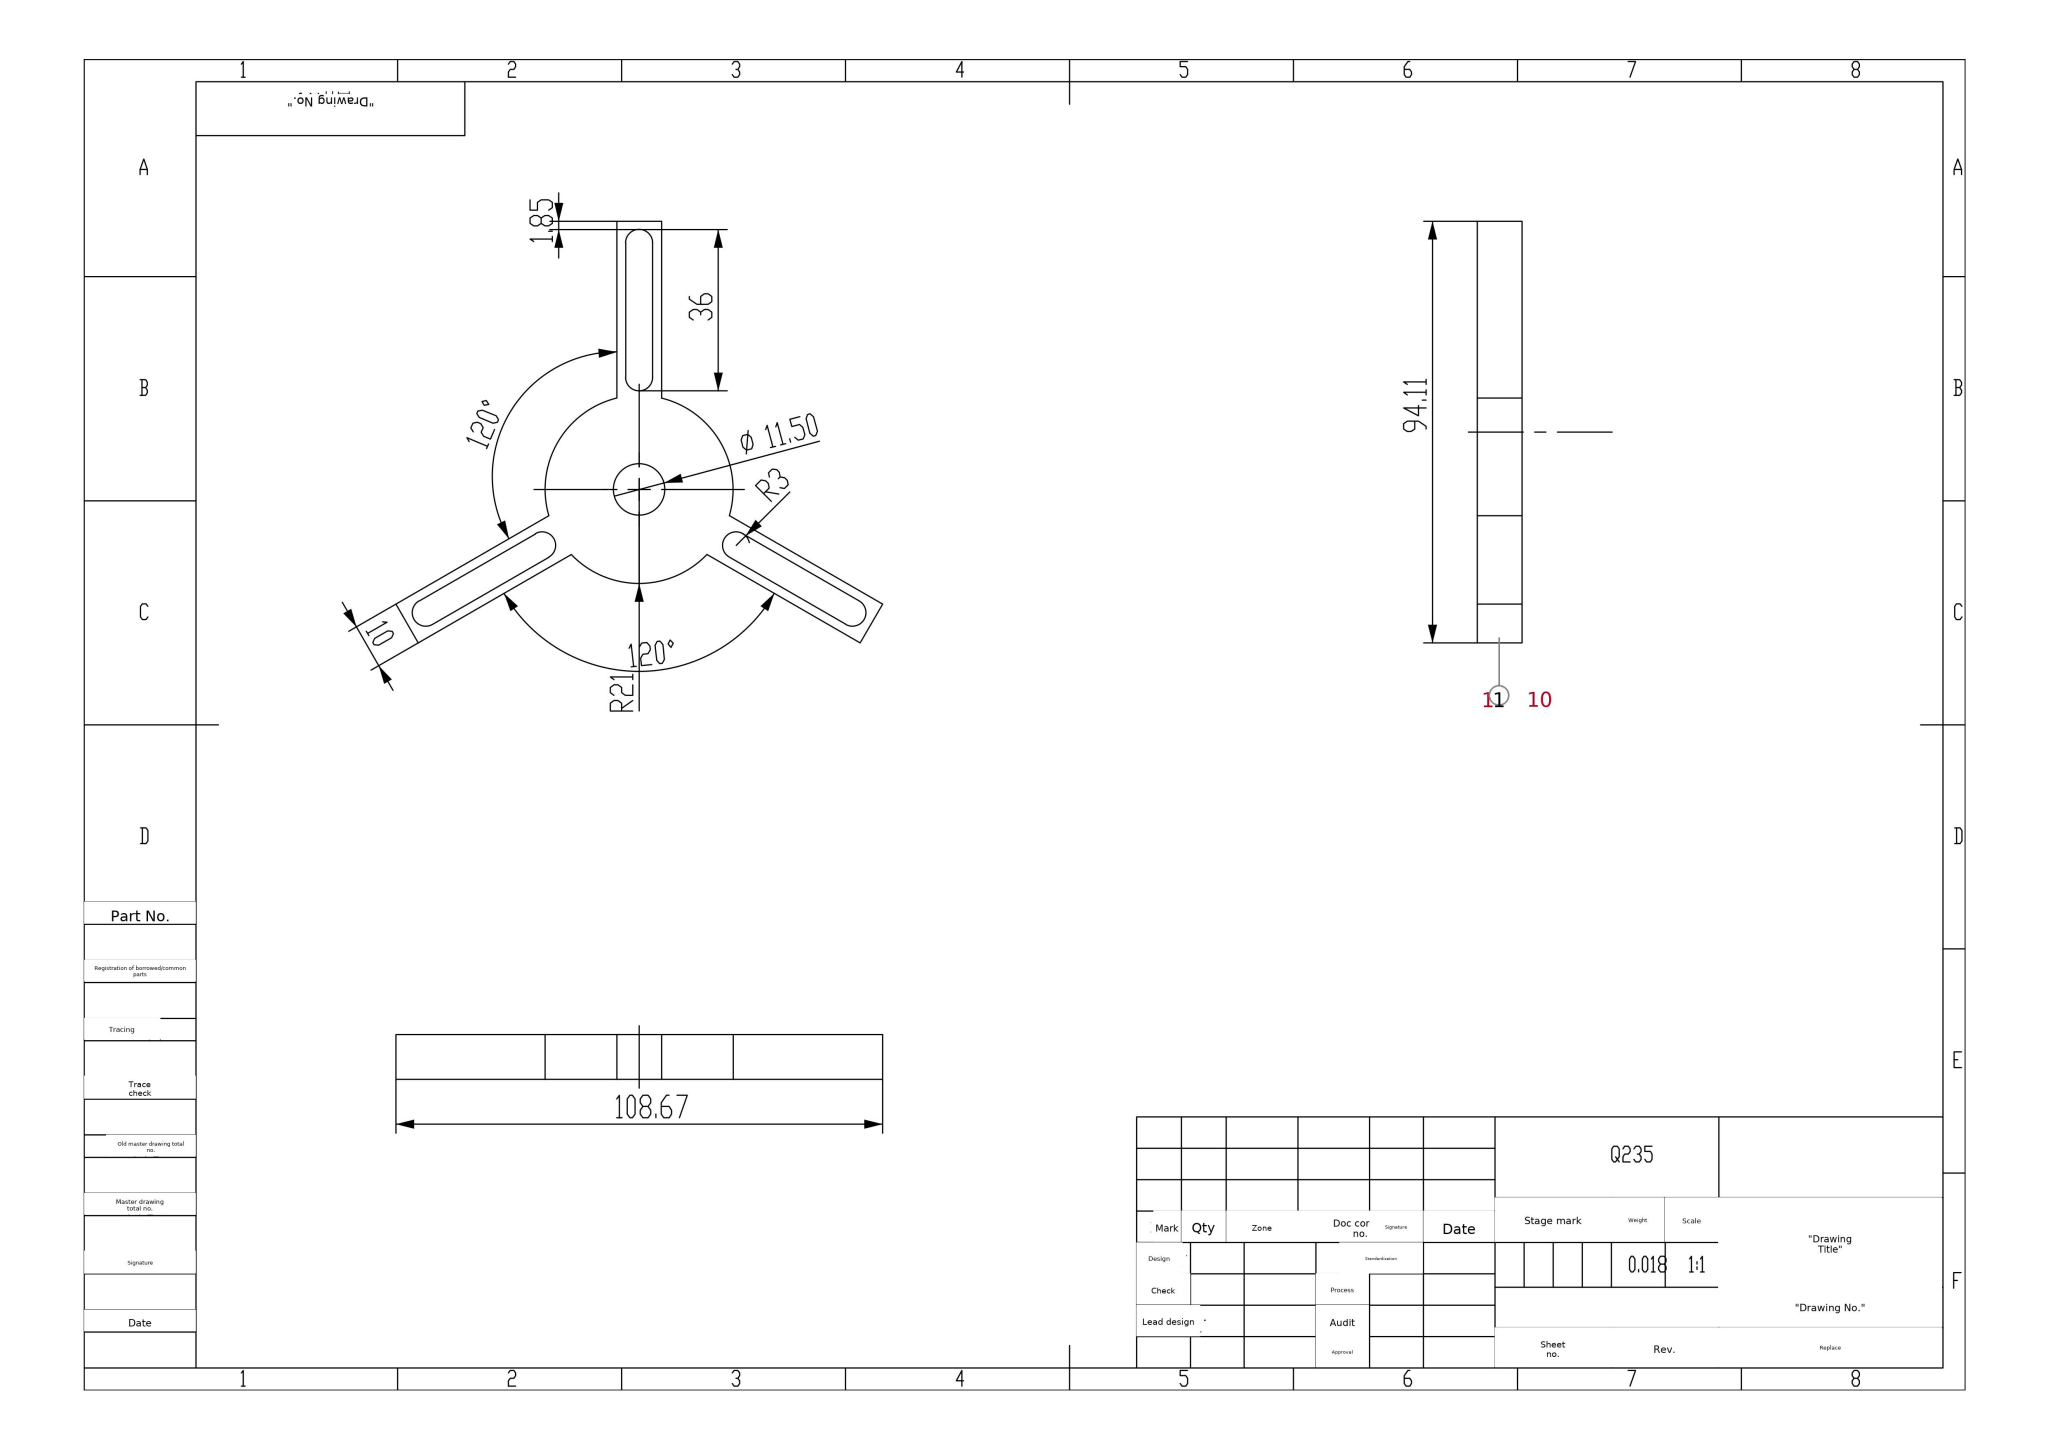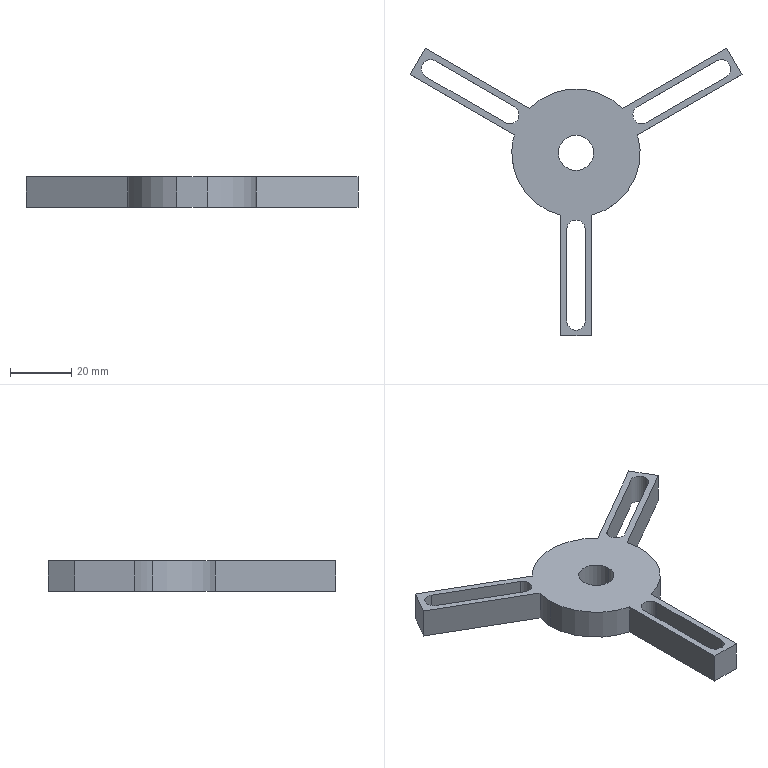Part | SolidWorks | mm | material Q235 | 1 solid | 31 faces | box 108.67 x 94.11 x 10 mm | volume 18283 mm3 | plane 17 | cylinder 14 | commonest cylinder face diameters 6 x8 42 x4 11.5 x2
build123d program:
from build123d import *

# Parameters (mm, degrees)
SKETCH1_R           = 21
SKETCH1_R_2         = 5.75
BOSS_EXTRUDE1_DEPTH = 10
BOSS_EXTRUDE2_DEPTH = 10
CUT_EXTRUDE1_DEPTH  = 65.213
CIRPATTERN1_COUNT   = 3


with BuildPart() as part:
    # Sketch1 → Boss-Extrude1 (new body)
    with BuildSketch(Plane.XY):
        Circle(SKETCH1_R)
        Circle(SKETCH1_R_2, mode=Mode.SUBTRACT)
    extrude(amount=BOSS_EXTRUDE1_DEPTH)

    # Sketch2 → Boss-Extrude2 (add)
    with BuildSketch(Plane(origin=(0, 0, 0), x_dir=(-1, 0, 0), z_dir=(0, 0, -1))):
        with BuildLine():
            ThreePointArc((5, -20.396), (0, -21), (-5, -20.396))
            Line((-5, -20.396), (-5, -59.853))
            Line((-5, -59.853), (5, -59.853))
            Line((5, -59.853), (5, -20.396))
        make_face()
    boss_extrude2 = extrude(amount=-BOSS_EXTRUDE2_DEPTH)

    # Sketch3 → Cut-Extrude1 (cut, through all)
    with BuildSketch(Plane(origin=(0, 0, 0), x_dir=(-1, 0, 0), z_dir=(0, 0, -1))):
        with BuildLine():
            Line((3, -25), (3, -55))
            ThreePointArc((3, -55), (0, -58), (-3, -55))
            Line((-3, -55), (-3, -25))
            ThreePointArc((-3, -25), (0, -22), (3, -25))
        make_face()
    cut_extrude1 = extrude(amount=-CUT_EXTRUDE1_DEPTH, mode=Mode.SUBTRACT)

    # CirPattern1: Boss-Extrude2, Cut-Extrude1 ×3 about axis
    cirpattern1_axis = Axis((0, 0, 0), (0, 0, 1))
    add([boss_extrude2.rotate(cirpattern1_axis, i * 360 / CIRPATTERN1_COUNT) for i in range(1, CIRPATTERN1_COUNT)])
    add([cut_extrude1.rotate(cirpattern1_axis, i * 360 / CIRPATTERN1_COUNT) for i in range(1, CIRPATTERN1_COUNT)], mode=Mode.SUBTRACT)


solid = part.part
STEP:
#1=CARTESIAN_POINT('',(-50.631,27.5,10.));
#2=VERTEX_POINT('',#1);
#3=CARTESIAN_POINT('',(-46.131,30.098,10.));
#4=VERTEX_POINT('',#3);
#5=CARTESIAN_POINT('',(-47.631,27.5,10.));
#6=DIRECTION('',(0.,0.,-1.));
#7=DIRECTION('',(0.5,0.866,0.));
#8=AXIS2_PLACEMENT_3D('',#5,#6,#7);
#9=CIRCLE('',#8,3.);
#10=EDGE_CURVE('',#2,#4,#9,.T.);
#11=ORIENTED_EDGE('',*,*,#10,.F.);
#12=CARTESIAN_POINT('',(-50.631,27.5,0.));
#13=VERTEX_POINT('',#12);
#14=CARTESIAN_POINT('',(-50.631,27.5,10.));
#15=DIRECTION('',(0.,0.,-1.));
#16=VECTOR('',#15,1000.);
#17=LINE('',#14,#16);
#18=EDGE_CURVE('',#2,#13,#17,.T.);
#19=ORIENTED_EDGE('',*,*,#18,.T.);
#20=CARTESIAN_POINT('',(-46.131,30.098,0.));
#21=VERTEX_POINT('',#20);
#22=CARTESIAN_POINT('',(-47.631,27.5,0.));
#23=DIRECTION('',(0.,0.,-1.));
#24=DIRECTION('',(0.5,0.866,0.));
#25=AXIS2_PLACEMENT_3D('',#22,#23,#24);
#26=CIRCLE('',#25,3.);
#27=EDGE_CURVE('',#13,#21,#26,.T.);
#28=ORIENTED_EDGE('',*,*,#27,.T.);
#29=CARTESIAN_POINT('',(-46.131,30.098,10.));
#30=DIRECTION('',(0.,0.,-1.));
#31=VECTOR('',#30,1000.);
#32=LINE('',#29,#31);
#33=EDGE_CURVE('',#4,#21,#32,.T.);
#34=ORIENTED_EDGE('',*,*,#33,.F.);
#35=EDGE_LOOP('',(#11,#19,#28,#34));
#36=FACE_OUTER_BOUND('',#35,.T.);
#37=CARTESIAN_POINT('',(-47.631,27.5,10.));
#38=DIRECTION('',(0.,0.,-1.));
#39=DIRECTION('',(-1.,0.,0.));
#40=AXIS2_PLACEMENT_3D('',#37,#38,#39);
#41=CYLINDRICAL_SURFACE('',#40,3.);
#42=ADVANCED_FACE('',(#36),#41,.F.);
#43=CARTESIAN_POINT('',(18.651,12.5,10.));
#44=VERTEX_POINT('',#43);
#45=CARTESIAN_POINT('',(20.151,15.098,10.));
#46=VERTEX_POINT('',#45);
#47=CARTESIAN_POINT('',(21.651,12.5,10.));
#48=DIRECTION('',(0.,0.,-1.));
#49=DIRECTION('',(0.5,-0.866,0.));
#50=AXIS2_PLACEMENT_3D('',#47,#48,#49);
#51=CIRCLE('',#50,3.);
#52=EDGE_CURVE('',#44,#46,#51,.T.);
#53=ORIENTED_EDGE('',*,*,#52,.F.);
#54=CARTESIAN_POINT('',(18.651,12.5,0.));
#55=VERTEX_POINT('',#54);
#56=CARTESIAN_POINT('',(18.651,12.5,10.));
#57=DIRECTION('',(0.,0.,-1.));
#58=VECTOR('',#57,1000.);
#59=LINE('',#56,#58);
#60=EDGE_CURVE('',#44,#55,#59,.T.);
#61=ORIENTED_EDGE('',*,*,#60,.T.);
#62=CARTESIAN_POINT('',(20.151,15.098,0.));
#63=VERTEX_POINT('',#62);
#64=CARTESIAN_POINT('',(21.651,12.5,0.));
#65=DIRECTION('',(0.,0.,-1.));
#66=DIRECTION('',(0.5,-0.866,0.));
#67=AXIS2_PLACEMENT_3D('',#64,#65,#66);
#68=CIRCLE('',#67,3.);
#69=EDGE_CURVE('',#55,#63,#68,.T.);
#70=ORIENTED_EDGE('',*,*,#69,.T.);
#71=CARTESIAN_POINT('',(20.151,15.098,10.));
#72=DIRECTION('',(0.,0.,-1.));
#73=VECTOR('',#72,1000.);
#74=LINE('',#71,#73);
#75=EDGE_CURVE('',#46,#63,#74,.T.);
#76=ORIENTED_EDGE('',*,*,#75,.F.);
#77=EDGE_LOOP('',(#53,#61,#70,#76));
#78=FACE_OUTER_BOUND('',#77,.T.);
#79=CARTESIAN_POINT('',(21.651,12.5,10.));
#80=DIRECTION('',(0.,0.,-1.));
#81=DIRECTION('',(-1.,0.,0.));
#82=AXIS2_PLACEMENT_3D('',#79,#80,#81);
#83=CYLINDRICAL_SURFACE('',#82,3.);
#84=ADVANCED_FACE('',(#78),#83,.F.);
#85=CARTESIAN_POINT('',(-5.75,0.,10.));
#86=VERTEX_POINT('',#85);
#87=CARTESIAN_POINT('',(5.75,0.,10.));
#88=VERTEX_POINT('',#87);
#89=CARTESIAN_POINT('',(0.,0.,10.));
#90=DIRECTION('',(0.,0.,1.));
#91=DIRECTION('',(1.,0.,0.));
#92=AXIS2_PLACEMENT_3D('',#89,#90,#91);
#93=CIRCLE('',#92,5.75);
#94=EDGE_CURVE('',#86,#88,#93,.T.);
#95=ORIENTED_EDGE('',*,*,#94,.T.);
#96=CARTESIAN_POINT('',(5.75,0.,0.));
#97=VERTEX_POINT('',#96);
#98=CARTESIAN_POINT('',(5.75,0.,10.));
#99=DIRECTION('',(0.,0.,-1.));
#100=VECTOR('',#99,1000.);
#101=LINE('',#98,#100);
#102=EDGE_CURVE('',#88,#97,#101,.T.);
#103=ORIENTED_EDGE('',*,*,#102,.T.);
#104=CARTESIAN_POINT('',(-5.75,0.,0.));
#105=VERTEX_POINT('',#104);
#106=CARTESIAN_POINT('',(0.,0.,0.));
#107=DIRECTION('',(0.,0.,1.));
#108=DIRECTION('',(1.,0.,0.));
#109=AXIS2_PLACEMENT_3D('',#106,#107,#108);
#110=CIRCLE('',#109,5.75);
#111=EDGE_CURVE('',#105,#97,#110,.T.);
#112=ORIENTED_EDGE('',*,*,#111,.F.);
#113=CARTESIAN_POINT('',(-5.75,0.,10.));
#114=DIRECTION('',(0.,0.,-1.));
#115=VECTOR('',#114,1000.);
#116=LINE('',#113,#115);
#117=EDGE_CURVE('',#86,#105,#116,.T.);
#118=ORIENTED_EDGE('',*,*,#117,.F.);
#119=EDGE_LOOP('',(#95,#103,#112,#118));
#120=FACE_OUTER_BOUND('',#119,.T.);
#121=CARTESIAN_POINT('',(0.,0.,10.));
#122=DIRECTION('',(0.,0.,-1.));
#123=DIRECTION('',(-1.,0.,0.));
#124=AXIS2_PLACEMENT_3D('',#121,#122,#123);
#125=CYLINDRICAL_SURFACE('',#124,5.75);
#126=ADVANCED_FACE('',(#120),#125,.F.);
#127=CARTESIAN_POINT('',(-21.,0.,10.));
#128=VERTEX_POINT('',#127);
#129=CARTESIAN_POINT('',(-5.,-20.396,10.));
#130=VERTEX_POINT('',#129);
#131=CARTESIAN_POINT('',(0.,0.,10.));
#132=DIRECTION('',(0.,0.,1.));
#133=DIRECTION('',(1.,0.,0.));
#134=AXIS2_PLACEMENT_3D('',#131,#132,#133);
#135=CIRCLE('',#134,21.);
#136=EDGE_CURVE('',#128,#130,#135,.T.);
#137=ORIENTED_EDGE('',*,*,#136,.F.);
#138=CARTESIAN_POINT('',(-21.,0.,0.));
#139=VERTEX_POINT('',#138);
#140=CARTESIAN_POINT('',(-21.,0.,10.));
#141=DIRECTION('',(0.,0.,-1.));
#142=VECTOR('',#141,1000.);
#143=LINE('',#140,#142);
#144=EDGE_CURVE('',#128,#139,#143,.T.);
#145=ORIENTED_EDGE('',*,*,#144,.T.);
#146=CARTESIAN_POINT('',(-5.,-20.396,0.));
#147=VERTEX_POINT('',#146);
#148=CARTESIAN_POINT('',(0.,0.,0.));
#149=DIRECTION('',(0.,0.,1.));
#150=DIRECTION('',(1.,0.,0.));
#151=AXIS2_PLACEMENT_3D('',#148,#149,#150);
#152=CIRCLE('',#151,21.);
#153=EDGE_CURVE('',#139,#147,#152,.T.);
#154=ORIENTED_EDGE('',*,*,#153,.T.);
#155=CARTESIAN_POINT('',(-5.,-20.396,10.));
#156=DIRECTION('',(0.,0.,-1.));
#157=VECTOR('',#156,1000.);
#158=LINE('',#155,#157);
#159=EDGE_CURVE('',#130,#147,#158,.T.);
#160=ORIENTED_EDGE('',*,*,#159,.F.);
#161=EDGE_LOOP('',(#137,#145,#154,#160));
#162=FACE_OUTER_BOUND('',#161,.T.);
#163=CARTESIAN_POINT('',(0.,0.,10.));
#164=DIRECTION('',(0.,0.,-1.));
#165=DIRECTION('',(-1.,0.,0.));
#166=AXIS2_PLACEMENT_3D('',#163,#164,#165);
#167=CYLINDRICAL_SURFACE('',#166,21.);
#168=ADVANCED_FACE('',(#162),#167,.T.);
#169=CARTESIAN_POINT('',(20.164,5.868,10.));
#170=VERTEX_POINT('',#169);
#171=CARTESIAN_POINT('',(20.164,5.868,0.));
#172=VERTEX_POINT('',#171);
#173=CARTESIAN_POINT('',(20.164,5.868,10.));
#174=DIRECTION('',(0.,0.,-1.));
#175=VECTOR('',#174,1000.);
#176=LINE('',#173,#175);
#177=EDGE_CURVE('',#170,#172,#176,.T.);
#178=ORIENTED_EDGE('',*,*,#177,.F.);
#179=CARTESIAN_POINT('',(5.,-20.396,10.));
#180=VERTEX_POINT('',#179);
#181=CARTESIAN_POINT('',(0.,0.,10.));
#182=DIRECTION('',(0.,0.,1.));
#183=DIRECTION('',(1.,0.,0.));
#184=AXIS2_PLACEMENT_3D('',#181,#182,#183);
#185=CIRCLE('',#184,21.);
#186=EDGE_CURVE('',#180,#170,#185,.T.);
#187=ORIENTED_EDGE('',*,*,#186,.F.);
#188=CARTESIAN_POINT('',(5.,-20.396,0.));
#189=VERTEX_POINT('',#188);
#190=CARTESIAN_POINT('',(5.,-20.396,10.));
#191=DIRECTION('',(0.,0.,-1.));
#192=VECTOR('',#191,1000.);
#193=LINE('',#190,#192);
#194=EDGE_CURVE('',#180,#189,#193,.T.);
#195=ORIENTED_EDGE('',*,*,#194,.T.);
#196=CARTESIAN_POINT('',(0.,0.,0.));
#197=DIRECTION('',(0.,0.,1.));
#198=DIRECTION('',(1.,0.,0.));
#199=AXIS2_PLACEMENT_3D('',#196,#197,#198);
#200=CIRCLE('',#199,21.);
#201=EDGE_CURVE('',#189,#172,#200,.T.);
#202=ORIENTED_EDGE('',*,*,#201,.T.);
#203=EDGE_LOOP('',(#178,#187,#195,#202));
#204=FACE_OUTER_BOUND('',#203,.T.);
#205=CARTESIAN_POINT('',(0.,0.,10.));
#206=DIRECTION('',(0.,0.,-1.));
#207=DIRECTION('',(-1.,0.,0.));
#208=AXIS2_PLACEMENT_3D('',#205,#206,#207);
#209=CYLINDRICAL_SURFACE('',#208,21.);
#210=ADVANCED_FACE('',(#204),#209,.T.);
#211=CARTESIAN_POINT('',(15.164,14.528,10.));
#212=VERTEX_POINT('',#211);
#213=CARTESIAN_POINT('',(-15.164,14.528,10.));
#214=VERTEX_POINT('',#213);
#215=CARTESIAN_POINT('',(0.,0.,10.));
#216=DIRECTION('',(0.,0.,1.));
#217=DIRECTION('',(1.,0.,0.));
#218=AXIS2_PLACEMENT_3D('',#215,#216,#217);
#219=CIRCLE('',#218,21.);
#220=EDGE_CURVE('',#212,#214,#219,.T.);
#221=ORIENTED_EDGE('',*,*,#220,.F.);
#222=CARTESIAN_POINT('',(15.164,14.528,0.));
#223=VERTEX_POINT('',#222);
#224=CARTESIAN_POINT('',(15.164,14.528,10.));
#225=DIRECTION('',(0.,0.,-1.));
#226=VECTOR('',#225,1000.);
#227=LINE('',#224,#226);
#228=EDGE_CURVE('',#212,#223,#227,.T.);
#229=ORIENTED_EDGE('',*,*,#228,.T.);
#230=CARTESIAN_POINT('',(-15.164,14.528,0.));
#231=VERTEX_POINT('',#230);
#232=CARTESIAN_POINT('',(0.,0.,0.));
#233=DIRECTION('',(0.,0.,1.));
#234=DIRECTION('',(1.,0.,0.));
#235=AXIS2_PLACEMENT_3D('',#232,#233,#234);
#236=CIRCLE('',#235,21.);
#237=EDGE_CURVE('',#223,#231,#236,.T.);
#238=ORIENTED_EDGE('',*,*,#237,.T.);
#239=CARTESIAN_POINT('',(-15.164,14.528,10.));
#240=DIRECTION('',(0.,0.,-1.));
#241=VECTOR('',#240,1000.);
#242=LINE('',#239,#241);
#243=EDGE_CURVE('',#214,#231,#242,.T.);
#244=ORIENTED_EDGE('',*,*,#243,.F.);
#245=EDGE_LOOP('',(#221,#229,#238,#244));
#246=FACE_OUTER_BOUND('',#245,.T.);
#247=CARTESIAN_POINT('',(0.,0.,10.));
#248=DIRECTION('',(0.,0.,-1.));
#249=DIRECTION('',(-1.,0.,0.));
#250=AXIS2_PLACEMENT_3D('',#247,#248,#249);
#251=CYLINDRICAL_SURFACE('',#250,21.);
#252=ADVANCED_FACE('',(#246),#251,.T.);
#253=ORIENTED_EDGE('',*,*,#144,.F.);
#254=CARTESIAN_POINT('',(-20.164,5.868,10.));
#255=VERTEX_POINT('',#254);
#256=CARTESIAN_POINT('',(0.,0.,10.));
#257=DIRECTION('',(0.,0.,1.));
#258=DIRECTION('',(1.,0.,0.));
#259=AXIS2_PLACEMENT_3D('',#256,#257,#258);
#260=CIRCLE('',#259,21.);
#261=EDGE_CURVE('',#255,#128,#260,.T.);
#262=ORIENTED_EDGE('',*,*,#261,.F.);
#263=CARTESIAN_POINT('',(-20.164,5.868,0.));
#264=VERTEX_POINT('',#263);
#265=CARTESIAN_POINT('',(-20.164,5.868,10.));
#266=DIRECTION('',(0.,0.,-1.));
#267=VECTOR('',#266,1000.);
#268=LINE('',#265,#267);
#269=EDGE_CURVE('',#255,#264,#268,.T.);
#270=ORIENTED_EDGE('',*,*,#269,.T.);
#271=CARTESIAN_POINT('',(0.,0.,0.));
#272=DIRECTION('',(0.,0.,1.));
#273=DIRECTION('',(1.,0.,0.));
#274=AXIS2_PLACEMENT_3D('',#271,#272,#273);
#275=CIRCLE('',#274,21.);
#276=EDGE_CURVE('',#264,#139,#275,.T.);
#277=ORIENTED_EDGE('',*,*,#276,.T.);
#278=EDGE_LOOP('',(#253,#262,#270,#277));
#279=FACE_OUTER_BOUND('',#278,.T.);
#280=CARTESIAN_POINT('',(0.,0.,10.));
#281=DIRECTION('',(0.,0.,-1.));
#282=DIRECTION('',(-1.,0.,0.));
#283=AXIS2_PLACEMENT_3D('',#280,#281,#282);
#284=CYLINDRICAL_SURFACE('',#283,21.);
#285=ADVANCED_FACE('',(#279),#284,.T.);
#286=CARTESIAN_POINT('',(-20.151,15.098,10.));
#287=VERTEX_POINT('',#286);
#288=CARTESIAN_POINT('',(-23.151,9.902,10.));
#289=VERTEX_POINT('',#288);
#290=CARTESIAN_POINT('',(-21.651,12.5,10.));
#291=DIRECTION('',(0.,0.,-1.));
#292=DIRECTION('',(0.5,0.866,0.));
#293=AXIS2_PLACEMENT_3D('',#290,#291,#292);
#294=CIRCLE('',#293,3.);
#295=EDGE_CURVE('',#287,#289,#294,.T.);
#296=ORIENTED_EDGE('',*,*,#295,.T.);
#297=CARTESIAN_POINT('',(-49.131,24.902,10.));
#298=VERTEX_POINT('',#297);
#299=CARTESIAN_POINT('',(-23.151,9.902,10.));
#300=DIRECTION('',(-0.866,0.5,0.));
#301=VECTOR('',#300,1000.);
#302=LINE('',#299,#301);
#303=EDGE_CURVE('',#289,#298,#302,.T.);
#304=ORIENTED_EDGE('',*,*,#303,.T.);
#305=CARTESIAN_POINT('',(-47.631,27.5,10.));
#306=DIRECTION('',(0.,0.,-1.));
#307=DIRECTION('',(0.5,0.866,0.));
#308=AXIS2_PLACEMENT_3D('',#305,#306,#307);
#309=CIRCLE('',#308,3.);
#310=EDGE_CURVE('',#298,#2,#309,.T.);
#311=ORIENTED_EDGE('',*,*,#310,.T.);
#312=ORIENTED_EDGE('',*,*,#10,.T.);
#313=CARTESIAN_POINT('',(-20.151,15.098,10.));
#314=DIRECTION('',(0.866,-0.5,0.));
#315=VECTOR('',#314,1000.);
#316=LINE('',#313,#315);
#317=EDGE_CURVE('',#4,#287,#316,.T.);
#318=ORIENTED_EDGE('',*,*,#317,.T.);
#319=EDGE_LOOP('',(#296,#304,#311,#312,#318));
#320=FACE_BOUND('',#319,.T.);
#321=CARTESIAN_POINT('',(23.151,9.902,10.));
#322=VERTEX_POINT('',#321);
#323=CARTESIAN_POINT('',(21.651,12.5,10.));
#324=DIRECTION('',(0.,0.,-1.));
#325=DIRECTION('',(0.5,-0.866,0.));
#326=AXIS2_PLACEMENT_3D('',#323,#324,#325);
#327=CIRCLE('',#326,3.);
#328=EDGE_CURVE('',#322,#44,#327,.T.);
#329=ORIENTED_EDGE('',*,*,#328,.T.);
#330=ORIENTED_EDGE('',*,*,#52,.T.);
#331=CARTESIAN_POINT('',(46.131,30.098,10.));
#332=VERTEX_POINT('',#331);
#333=CARTESIAN_POINT('',(20.151,15.098,10.));
#334=DIRECTION('',(0.866,0.5,0.));
#335=VECTOR('',#334,1000.);
#336=LINE('',#333,#335);
#337=EDGE_CURVE('',#46,#332,#336,.T.);
#338=ORIENTED_EDGE('',*,*,#337,.T.);
#339=CARTESIAN_POINT('',(49.131,24.902,10.));
#340=VERTEX_POINT('',#339);
#341=CARTESIAN_POINT('',(47.631,27.5,10.));
#342=DIRECTION('',(0.,0.,-1.));
#343=DIRECTION('',(0.5,-0.866,0.));
#344=AXIS2_PLACEMENT_3D('',#341,#342,#343);
#345=CIRCLE('',#344,3.);
#346=EDGE_CURVE('',#332,#340,#345,.T.);
#347=ORIENTED_EDGE('',*,*,#346,.T.);
#348=CARTESIAN_POINT('',(23.151,9.902,10.));
#349=DIRECTION('',(-0.866,-0.5,0.));
#350=VECTOR('',#349,1000.);
#351=LINE('',#348,#350);
#352=EDGE_CURVE('',#340,#322,#351,.T.);
#353=ORIENTED_EDGE('',*,*,#352,.T.);
#354=EDGE_LOOP('',(#329,#330,#338,#347,#353));
#355=FACE_BOUND('',#354,.T.);
#356=CARTESIAN_POINT('',(-3.,-25.,10.));
#357=VERTEX_POINT('',#356);
#358=CARTESIAN_POINT('',(3.,-25.,10.));
#359=VERTEX_POINT('',#358);
#360=CARTESIAN_POINT('',(-0.,-25.,10.));
#361=DIRECTION('',(0.,0.,-1.));
#362=DIRECTION('',(-1.,0.,0.));
#363=AXIS2_PLACEMENT_3D('',#360,#361,#362);
#364=CIRCLE('',#363,3.);
#365=EDGE_CURVE('',#357,#359,#364,.T.);
#366=ORIENTED_EDGE('',*,*,#365,.T.);
#367=CARTESIAN_POINT('',(3.,-55.,10.));
#368=VERTEX_POINT('',#367);
#369=CARTESIAN_POINT('',(3.,-25.,10.));
#370=DIRECTION('',(-0.,-1.,0.));
#371=VECTOR('',#370,1000.);
#372=LINE('',#369,#371);
#373=EDGE_CURVE('',#359,#368,#372,.T.);
#374=ORIENTED_EDGE('',*,*,#373,.T.);
#375=CARTESIAN_POINT('',(-3.,-55.,10.));
#376=VERTEX_POINT('',#375);
#377=CARTESIAN_POINT('',(-0.,-55.,10.));
#378=DIRECTION('',(0.,0.,-1.));
#379=DIRECTION('',(-1.,0.,0.));
#380=AXIS2_PLACEMENT_3D('',#377,#378,#379);
#381=CIRCLE('',#380,3.);
#382=EDGE_CURVE('',#368,#376,#381,.T.);
#383=ORIENTED_EDGE('',*,*,#382,.T.);
#384=CARTESIAN_POINT('',(-3.,-25.,10.));
#385=DIRECTION('',(0.,1.,0.));
#386=VECTOR('',#385,1000.);
#387=LINE('',#384,#386);
#388=EDGE_CURVE('',#376,#357,#387,.T.);
#389=ORIENTED_EDGE('',*,*,#388,.T.);
#390=EDGE_LOOP('',(#366,#374,#383,#389));
#391=FACE_BOUND('',#390,.T.);
#392=ORIENTED_EDGE('',*,*,#186,.T.);
#393=CARTESIAN_POINT('',(54.334,25.596,10.));
#394=VERTEX_POINT('',#393);
#395=CARTESIAN_POINT('',(2.5,-4.33,10.));
#396=DIRECTION('',(0.866,0.5,0.));
#397=VECTOR('',#396,1000.);
#398=LINE('',#395,#397);
#399=EDGE_CURVE('',#170,#394,#398,.T.);
#400=ORIENTED_EDGE('',*,*,#399,.T.);
#401=CARTESIAN_POINT('',(49.334,34.256,10.));
#402=VERTEX_POINT('',#401);
#403=CARTESIAN_POINT('',(51.834,29.926,10.));
#404=DIRECTION('',(0.5,-0.866,0.));
#405=VECTOR('',#404,1000.);
#406=LINE('',#403,#405);
#407=EDGE_CURVE('',#402,#394,#406,.T.);
#408=ORIENTED_EDGE('',*,*,#407,.F.);
#409=CARTESIAN_POINT('',(-2.5,4.33,10.));
#410=DIRECTION('',(0.866,0.5,0.));
#411=VECTOR('',#410,1000.);
#412=LINE('',#409,#411);
#413=EDGE_CURVE('',#212,#402,#412,.T.);
#414=ORIENTED_EDGE('',*,*,#413,.F.);
#415=ORIENTED_EDGE('',*,*,#220,.T.);
#416=CARTESIAN_POINT('',(-49.334,34.256,10.));
#417=VERTEX_POINT('',#416);
#418=CARTESIAN_POINT('',(2.5,4.33,10.));
#419=DIRECTION('',(-0.866,0.5,0.));
#420=VECTOR('',#419,1000.);
#421=LINE('',#418,#420);
#422=EDGE_CURVE('',#214,#417,#421,.T.);
#423=ORIENTED_EDGE('',*,*,#422,.T.);
#424=CARTESIAN_POINT('',(-54.334,25.596,10.));
#425=VERTEX_POINT('',#424);
#426=CARTESIAN_POINT('',(-51.834,29.926,10.));
#427=DIRECTION('',(0.5,0.866,0.));
#428=VECTOR('',#427,1000.);
#429=LINE('',#426,#428);
#430=EDGE_CURVE('',#425,#417,#429,.T.);
#431=ORIENTED_EDGE('',*,*,#430,.F.);
#432=CARTESIAN_POINT('',(-2.5,-4.33,10.));
#433=DIRECTION('',(-0.866,0.5,0.));
#434=VECTOR('',#433,1000.);
#435=LINE('',#432,#434);
#436=EDGE_CURVE('',#255,#425,#435,.T.);
#437=ORIENTED_EDGE('',*,*,#436,.F.);
#438=ORIENTED_EDGE('',*,*,#261,.T.);
#439=ORIENTED_EDGE('',*,*,#136,.T.);
#440=CARTESIAN_POINT('',(-5.,-59.853,10.));
#441=VERTEX_POINT('',#440);
#442=CARTESIAN_POINT('',(-5.,0.,10.));
#443=DIRECTION('',(0.,-1.,0.));
#444=VECTOR('',#443,1000.);
#445=LINE('',#442,#444);
#446=EDGE_CURVE('',#130,#441,#445,.T.);
#447=ORIENTED_EDGE('',*,*,#446,.T.);
#448=CARTESIAN_POINT('',(5.,-59.853,10.));
#449=VERTEX_POINT('',#448);
#450=CARTESIAN_POINT('',(0.,-59.853,10.));
#451=DIRECTION('',(-1.,0.,0.));
#452=VECTOR('',#451,1000.);
#453=LINE('',#450,#452);
#454=EDGE_CURVE('',#449,#441,#453,.T.);
#455=ORIENTED_EDGE('',*,*,#454,.F.);
#456=CARTESIAN_POINT('',(5.,0.,10.));
#457=DIRECTION('',(0.,-1.,0.));
#458=VECTOR('',#457,1000.);
#459=LINE('',#456,#458);
#460=EDGE_CURVE('',#180,#449,#459,.T.);
#461=ORIENTED_EDGE('',*,*,#460,.F.);
#462=EDGE_LOOP('',(#392,#400,#408,#414,#415,#423,#431,#437,#438,#439,#447,#455,#461));
#463=FACE_OUTER_BOUND('',#462,.T.);
#464=ORIENTED_EDGE('',*,*,#94,.F.);
#465=CARTESIAN_POINT('',(0.,0.,10.));
#466=DIRECTION('',(0.,0.,1.));
#467=DIRECTION('',(1.,0.,0.));
#468=AXIS2_PLACEMENT_3D('',#465,#466,#467);
#469=CIRCLE('',#468,5.75);
#470=EDGE_CURVE('',#88,#86,#469,.T.);
#471=ORIENTED_EDGE('',*,*,#470,.F.);
#472=EDGE_LOOP('',(#464,#471));
#473=FACE_BOUND('',#472,.T.);
#474=CARTESIAN_POINT('',(0.,0.,10.));
#475=DIRECTION('',(0.,0.,1.));
#476=DIRECTION('',(1.,0.,0.));
#477=AXIS2_PLACEMENT_3D('',#474,#475,#476);
#478=PLANE('',#477);
#479=ADVANCED_FACE('',(#320,#355,#391,#463,#473),#478,.T.);
#480=CARTESIAN_POINT('',(-23.151,9.902,0.));
#481=VERTEX_POINT('',#480);
#482=CARTESIAN_POINT('',(-49.131,24.902,0.));
#483=VERTEX_POINT('',#482);
#484=CARTESIAN_POINT('',(-23.151,9.902,0.));
#485=DIRECTION('',(-0.866,0.5,0.));
#486=VECTOR('',#485,1000.);
#487=LINE('',#484,#486);
#488=EDGE_CURVE('',#481,#483,#487,.T.);
#489=ORIENTED_EDGE('',*,*,#488,.F.);
#490=CARTESIAN_POINT('',(-20.151,15.098,0.));
#491=VERTEX_POINT('',#490);
#492=CARTESIAN_POINT('',(-21.651,12.5,0.));
#493=DIRECTION('',(0.,0.,-1.));
#494=DIRECTION('',(0.5,0.866,0.));
#495=AXIS2_PLACEMENT_3D('',#492,#493,#494);
#496=CIRCLE('',#495,3.);
#497=EDGE_CURVE('',#491,#481,#496,.T.);
#498=ORIENTED_EDGE('',*,*,#497,.F.);
#499=CARTESIAN_POINT('',(-20.151,15.098,0.));
#500=DIRECTION('',(0.866,-0.5,0.));
#501=VECTOR('',#500,1000.);
#502=LINE('',#499,#501);
#503=EDGE_CURVE('',#21,#491,#502,.T.);
#504=ORIENTED_EDGE('',*,*,#503,.F.);
#505=ORIENTED_EDGE('',*,*,#27,.F.);
#506=CARTESIAN_POINT('',(-47.631,27.5,0.));
#507=DIRECTION('',(0.,0.,-1.));
#508=DIRECTION('',(0.5,0.866,0.));
#509=AXIS2_PLACEMENT_3D('',#506,#507,#508);
#510=CIRCLE('',#509,3.);
#511=EDGE_CURVE('',#483,#13,#510,.T.);
#512=ORIENTED_EDGE('',*,*,#511,.F.);
#513=EDGE_LOOP('',(#489,#498,#504,#505,#512));
#514=FACE_BOUND('',#513,.T.);
#515=CARTESIAN_POINT('',(46.131,30.098,0.));
#516=VERTEX_POINT('',#515);
#517=CARTESIAN_POINT('',(20.151,15.098,0.));
#518=DIRECTION('',(0.866,0.5,0.));
#519=VECTOR('',#518,1000.);
#520=LINE('',#517,#519);
#521=EDGE_CURVE('',#63,#516,#520,.T.);
#522=ORIENTED_EDGE('',*,*,#521,.F.);
#523=ORIENTED_EDGE('',*,*,#69,.F.);
#524=CARTESIAN_POINT('',(23.151,9.902,0.));
#525=VERTEX_POINT('',#524);
#526=CARTESIAN_POINT('',(21.651,12.5,0.));
#527=DIRECTION('',(0.,0.,-1.));
#528=DIRECTION('',(0.5,-0.866,0.));
#529=AXIS2_PLACEMENT_3D('',#526,#527,#528);
#530=CIRCLE('',#529,3.);
#531=EDGE_CURVE('',#525,#55,#530,.T.);
#532=ORIENTED_EDGE('',*,*,#531,.F.);
#533=CARTESIAN_POINT('',(49.131,24.902,0.));
#534=VERTEX_POINT('',#533);
#535=CARTESIAN_POINT('',(23.151,9.902,0.));
#536=DIRECTION('',(-0.866,-0.5,0.));
#537=VECTOR('',#536,1000.);
#538=LINE('',#535,#537);
#539=EDGE_CURVE('',#534,#525,#538,.T.);
#540=ORIENTED_EDGE('',*,*,#539,.F.);
#541=CARTESIAN_POINT('',(47.631,27.5,0.));
#542=DIRECTION('',(0.,0.,-1.));
#543=DIRECTION('',(0.5,-0.866,0.));
#544=AXIS2_PLACEMENT_3D('',#541,#542,#543);
#545=CIRCLE('',#544,3.);
#546=EDGE_CURVE('',#516,#534,#545,.T.);
#547=ORIENTED_EDGE('',*,*,#546,.F.);
#548=EDGE_LOOP('',(#522,#523,#532,#540,#547));
#549=FACE_BOUND('',#548,.T.);
#550=CARTESIAN_POINT('',(3.,-25.,0.));
#551=VERTEX_POINT('',#550);
#552=CARTESIAN_POINT('',(3.,-55.,0.));
#553=VERTEX_POINT('',#552);
#554=CARTESIAN_POINT('',(3.,-25.,0.));
#555=DIRECTION('',(-0.,-1.,0.));
#556=VECTOR('',#555,1000.);
#557=LINE('',#554,#556);
#558=EDGE_CURVE('',#551,#553,#557,.T.);
#559=ORIENTED_EDGE('',*,*,#558,.F.);
#560=CARTESIAN_POINT('',(-3.,-25.,0.));
#561=VERTEX_POINT('',#560);
#562=CARTESIAN_POINT('',(-0.,-25.,0.));
#563=DIRECTION('',(0.,0.,-1.));
#564=DIRECTION('',(-1.,0.,0.));
#565=AXIS2_PLACEMENT_3D('',#562,#563,#564);
#566=CIRCLE('',#565,3.);
#567=EDGE_CURVE('',#561,#551,#566,.T.);
#568=ORIENTED_EDGE('',*,*,#567,.F.);
#569=CARTESIAN_POINT('',(-3.,-55.,0.));
#570=VERTEX_POINT('',#569);
#571=CARTESIAN_POINT('',(-3.,-25.,0.));
#572=DIRECTION('',(0.,1.,0.));
#573=VECTOR('',#572,1000.);
#574=LINE('',#571,#573);
#575=EDGE_CURVE('',#570,#561,#574,.T.);
#576=ORIENTED_EDGE('',*,*,#575,.F.);
#577=CARTESIAN_POINT('',(-0.,-55.,0.));
#578=DIRECTION('',(0.,0.,-1.));
#579=DIRECTION('',(-1.,0.,0.));
#580=AXIS2_PLACEMENT_3D('',#577,#578,#579);
#581=CIRCLE('',#580,3.);
#582=EDGE_CURVE('',#553,#570,#581,.T.);
#583=ORIENTED_EDGE('',*,*,#582,.F.);
#584=EDGE_LOOP('',(#559,#568,#576,#583));
#585=FACE_BOUND('',#584,.T.);
#586=ORIENTED_EDGE('',*,*,#201,.F.);
#587=CARTESIAN_POINT('',(5.,-59.853,0.));
#588=VERTEX_POINT('',#587);
#589=CARTESIAN_POINT('',(5.,0.,0.));
#590=DIRECTION('',(0.,-1.,0.));
#591=VECTOR('',#590,1000.);
#592=LINE('',#589,#591);
#593=EDGE_CURVE('',#189,#588,#592,.T.);
#594=ORIENTED_EDGE('',*,*,#593,.T.);
#595=CARTESIAN_POINT('',(-5.,-59.853,0.));
#596=VERTEX_POINT('',#595);
#597=CARTESIAN_POINT('',(0.,-59.853,0.));
#598=DIRECTION('',(-1.,0.,0.));
#599=VECTOR('',#598,1000.);
#600=LINE('',#597,#599);
#601=EDGE_CURVE('',#588,#596,#600,.T.);
#602=ORIENTED_EDGE('',*,*,#601,.T.);
#603=CARTESIAN_POINT('',(-5.,0.,0.));
#604=DIRECTION('',(0.,-1.,0.));
#605=VECTOR('',#604,1000.);
#606=LINE('',#603,#605);
#607=EDGE_CURVE('',#147,#596,#606,.T.);
#608=ORIENTED_EDGE('',*,*,#607,.F.);
#609=ORIENTED_EDGE('',*,*,#153,.F.);
#610=ORIENTED_EDGE('',*,*,#276,.F.);
#611=CARTESIAN_POINT('',(-54.334,25.596,0.));
#612=VERTEX_POINT('',#611);
#613=CARTESIAN_POINT('',(-2.5,-4.33,0.));
#614=DIRECTION('',(-0.866,0.5,0.));
#615=VECTOR('',#614,1000.);
#616=LINE('',#613,#615);
#617=EDGE_CURVE('',#264,#612,#616,.T.);
#618=ORIENTED_EDGE('',*,*,#617,.T.);
#619=CARTESIAN_POINT('',(-49.334,34.256,0.));
#620=VERTEX_POINT('',#619);
#621=CARTESIAN_POINT('',(-51.834,29.926,0.));
#622=DIRECTION('',(0.5,0.866,0.));
#623=VECTOR('',#622,1000.);
#624=LINE('',#621,#623);
#625=EDGE_CURVE('',#612,#620,#624,.T.);
#626=ORIENTED_EDGE('',*,*,#625,.T.);
#627=CARTESIAN_POINT('',(2.5,4.33,0.));
#628=DIRECTION('',(-0.866,0.5,0.));
#629=VECTOR('',#628,1000.);
#630=LINE('',#627,#629);
#631=EDGE_CURVE('',#231,#620,#630,.T.);
#632=ORIENTED_EDGE('',*,*,#631,.F.);
#633=ORIENTED_EDGE('',*,*,#237,.F.);
#634=CARTESIAN_POINT('',(49.334,34.256,0.));
#635=VERTEX_POINT('',#634);
#636=CARTESIAN_POINT('',(-2.5,4.33,0.));
#637=DIRECTION('',(0.866,0.5,0.));
#638=VECTOR('',#637,1000.);
#639=LINE('',#636,#638);
#640=EDGE_CURVE('',#223,#635,#639,.T.);
#641=ORIENTED_EDGE('',*,*,#640,.T.);
#642=CARTESIAN_POINT('',(54.334,25.596,0.));
#643=VERTEX_POINT('',#642);
#644=CARTESIAN_POINT('',(51.834,29.926,0.));
#645=DIRECTION('',(0.5,-0.866,0.));
#646=VECTOR('',#645,1000.);
#647=LINE('',#644,#646);
#648=EDGE_CURVE('',#635,#643,#647,.T.);
#649=ORIENTED_EDGE('',*,*,#648,.T.);
#650=CARTESIAN_POINT('',(2.5,-4.33,0.));
#651=DIRECTION('',(0.866,0.5,0.));
#652=VECTOR('',#651,1000.);
#653=LINE('',#650,#652);
#654=EDGE_CURVE('',#172,#643,#653,.T.);
#655=ORIENTED_EDGE('',*,*,#654,.F.);
#656=EDGE_LOOP('',(#586,#594,#602,#608,#609,#610,#618,#626,#632,#633,#641,#649,#655));
#657=FACE_OUTER_BOUND('',#656,.T.);
#658=ORIENTED_EDGE('',*,*,#111,.T.);
#659=CARTESIAN_POINT('',(0.,0.,0.));
#660=DIRECTION('',(0.,0.,1.));
#661=DIRECTION('',(1.,0.,0.));
#662=AXIS2_PLACEMENT_3D('',#659,#660,#661);
#663=CIRCLE('',#662,5.75);
#664=EDGE_CURVE('',#97,#105,#663,.T.);
#665=ORIENTED_EDGE('',*,*,#664,.T.);
#666=EDGE_LOOP('',(#658,#665));
#667=FACE_BOUND('',#666,.T.);
#668=CARTESIAN_POINT('',(0.,0.,0.));
#669=DIRECTION('',(0.,0.,1.));
#670=DIRECTION('',(1.,0.,0.));
#671=AXIS2_PLACEMENT_3D('',#668,#669,#670);
#672=PLANE('',#671);
#673=ADVANCED_FACE('',(#514,#549,#585,#657,#667),#672,.F.);
#674=ORIENTED_EDGE('',*,*,#102,.F.);
#675=ORIENTED_EDGE('',*,*,#470,.T.);
#676=ORIENTED_EDGE('',*,*,#117,.T.);
#677=ORIENTED_EDGE('',*,*,#664,.F.);
#678=EDGE_LOOP('',(#674,#675,#676,#677));
#679=FACE_OUTER_BOUND('',#678,.T.);
#680=CARTESIAN_POINT('',(0.,0.,10.));
#681=DIRECTION('',(0.,0.,-1.));
#682=DIRECTION('',(-1.,0.,0.));
#683=AXIS2_PLACEMENT_3D('',#680,#681,#682);
#684=CYLINDRICAL_SURFACE('',#683,5.75);
#685=ADVANCED_FACE('',(#679),#684,.F.);
#686=ORIENTED_EDGE('',*,*,#607,.T.);
#687=CARTESIAN_POINT('',(-5.,-59.853,10.));
#688=DIRECTION('',(0.,0.,-1.));
#689=VECTOR('',#688,1000.);
#690=LINE('',#687,#689);
#691=EDGE_CURVE('',#441,#596,#690,.T.);
#692=ORIENTED_EDGE('',*,*,#691,.F.);
#693=ORIENTED_EDGE('',*,*,#446,.F.);
#694=ORIENTED_EDGE('',*,*,#159,.T.);
#695=EDGE_LOOP('',(#686,#692,#693,#694));
#696=FACE_OUTER_BOUND('',#695,.T.);
#697=CARTESIAN_POINT('',(-5.,0.,10.));
#698=DIRECTION('',(1.,0.,0.));
#699=DIRECTION('',(0.,0.,-1.));
#700=AXIS2_PLACEMENT_3D('',#697,#698,#699);
#701=PLANE('',#700);
#702=ADVANCED_FACE('',(#696),#701,.F.);
#703=ORIENTED_EDGE('',*,*,#601,.F.);
#704=CARTESIAN_POINT('',(5.,-59.853,10.));
#705=DIRECTION('',(0.,0.,-1.));
#706=VECTOR('',#705,1000.);
#707=LINE('',#704,#706);
#708=EDGE_CURVE('',#449,#588,#707,.T.);
#709=ORIENTED_EDGE('',*,*,#708,.F.);
#710=ORIENTED_EDGE('',*,*,#454,.T.);
#711=ORIENTED_EDGE('',*,*,#691,.T.);
#712=EDGE_LOOP('',(#703,#709,#710,#711));
#713=FACE_OUTER_BOUND('',#712,.T.);
#714=CARTESIAN_POINT('',(0.,-59.853,10.));
#715=DIRECTION('',(0.,-1.,0.));
#716=DIRECTION('',(0.,0.,-1.));
#717=AXIS2_PLACEMENT_3D('',#714,#715,#716);
#718=PLANE('',#717);
#719=ADVANCED_FACE('',(#713),#718,.T.);
#720=ORIENTED_EDGE('',*,*,#593,.F.);
#721=ORIENTED_EDGE('',*,*,#194,.F.);
#722=ORIENTED_EDGE('',*,*,#460,.T.);
#723=ORIENTED_EDGE('',*,*,#708,.T.);
#724=EDGE_LOOP('',(#720,#721,#722,#723));
#725=FACE_OUTER_BOUND('',#724,.T.);
#726=CARTESIAN_POINT('',(5.,0.,10.));
#727=DIRECTION('',(1.,0.,0.));
#728=DIRECTION('',(0.,0.,-1.));
#729=AXIS2_PLACEMENT_3D('',#726,#727,#728);
#730=PLANE('',#729);
#731=ADVANCED_FACE('',(#725),#730,.T.);
#732=ORIENTED_EDGE('',*,*,#567,.T.);
#733=CARTESIAN_POINT('',(3.,-25.,10.));
#734=DIRECTION('',(0.,0.,-1.));
#735=VECTOR('',#734,1000.);
#736=LINE('',#733,#735);
#737=EDGE_CURVE('',#359,#551,#736,.T.);
#738=ORIENTED_EDGE('',*,*,#737,.F.);
#739=ORIENTED_EDGE('',*,*,#365,.F.);
#740=CARTESIAN_POINT('',(-3.,-25.,10.));
#741=DIRECTION('',(0.,0.,-1.));
#742=VECTOR('',#741,1000.);
#743=LINE('',#740,#742);
#744=EDGE_CURVE('',#357,#561,#743,.T.);
#745=ORIENTED_EDGE('',*,*,#744,.T.);
#746=EDGE_LOOP('',(#732,#738,#739,#745));
#747=FACE_OUTER_BOUND('',#746,.T.);
#748=CARTESIAN_POINT('',(-0.,-25.,10.));
#749=DIRECTION('',(0.,0.,-1.));
#750=DIRECTION('',(-1.,0.,0.));
#751=AXIS2_PLACEMENT_3D('',#748,#749,#750);
#752=CYLINDRICAL_SURFACE('',#751,3.);
#753=ADVANCED_FACE('',(#747),#752,.F.);
#754=ORIENTED_EDGE('',*,*,#575,.T.);
#755=ORIENTED_EDGE('',*,*,#744,.F.);
#756=ORIENTED_EDGE('',*,*,#388,.F.);
#757=CARTESIAN_POINT('',(-3.,-55.,10.));
#758=DIRECTION('',(0.,0.,-1.));
#759=VECTOR('',#758,1000.);
#760=LINE('',#757,#759);
#761=EDGE_CURVE('',#376,#570,#760,.T.);
#762=ORIENTED_EDGE('',*,*,#761,.T.);
#763=EDGE_LOOP('',(#754,#755,#756,#762));
#764=FACE_OUTER_BOUND('',#763,.T.);
#765=CARTESIAN_POINT('',(-3.,-25.,10.));
#766=DIRECTION('',(-1.,0.,0.));
#767=DIRECTION('',(-0.,-1.,0.));
#768=AXIS2_PLACEMENT_3D('',#765,#766,#767);
#769=PLANE('',#768);
#770=ADVANCED_FACE('',(#764),#769,.F.);
#771=ORIENTED_EDGE('',*,*,#582,.T.);
#772=ORIENTED_EDGE('',*,*,#761,.F.);
#773=ORIENTED_EDGE('',*,*,#382,.F.);
#774=CARTESIAN_POINT('',(3.,-55.,10.));
#775=DIRECTION('',(0.,0.,-1.));
#776=VECTOR('',#775,1000.);
#777=LINE('',#774,#776);
#778=EDGE_CURVE('',#368,#553,#777,.T.);
#779=ORIENTED_EDGE('',*,*,#778,.T.);
#780=EDGE_LOOP('',(#771,#772,#773,#779));
#781=FACE_OUTER_BOUND('',#780,.T.);
#782=CARTESIAN_POINT('',(-0.,-55.,10.));
#783=DIRECTION('',(0.,0.,-1.));
#784=DIRECTION('',(-1.,0.,0.));
#785=AXIS2_PLACEMENT_3D('',#782,#783,#784);
#786=CYLINDRICAL_SURFACE('',#785,3.);
#787=ADVANCED_FACE('',(#781),#786,.F.);
#788=ORIENTED_EDGE('',*,*,#558,.T.);
#789=ORIENTED_EDGE('',*,*,#778,.F.);
#790=ORIENTED_EDGE('',*,*,#373,.F.);
#791=ORIENTED_EDGE('',*,*,#737,.T.);
#792=EDGE_LOOP('',(#788,#789,#790,#791));
#793=FACE_OUTER_BOUND('',#792,.T.);
#794=CARTESIAN_POINT('',(3.,-25.,10.));
#795=DIRECTION('',(1.,-0.,0.));
#796=DIRECTION('',(0.,1.,0.));
#797=AXIS2_PLACEMENT_3D('',#794,#795,#796);
#798=PLANE('',#797);
#799=ADVANCED_FACE('',(#793),#798,.F.);
#800=ORIENTED_EDGE('',*,*,#631,.T.);
#801=CARTESIAN_POINT('',(-49.334,34.256,10.));
#802=DIRECTION('',(0.,0.,-1.));
#803=VECTOR('',#802,1000.);
#804=LINE('',#801,#803);
#805=EDGE_CURVE('',#417,#620,#804,.T.);
#806=ORIENTED_EDGE('',*,*,#805,.F.);
#807=ORIENTED_EDGE('',*,*,#422,.F.);
#808=ORIENTED_EDGE('',*,*,#243,.T.);
#809=EDGE_LOOP('',(#800,#806,#807,#808));
#810=FACE_OUTER_BOUND('',#809,.T.);
#811=CARTESIAN_POINT('',(2.5,4.33,10.));
#812=DIRECTION('',(-0.5,-0.866,0.));
#813=DIRECTION('',(0.866,-0.5,0.));
#814=AXIS2_PLACEMENT_3D('',#811,#812,#813);
#815=PLANE('',#814);
#816=ADVANCED_FACE('',(#810),#815,.F.);
#817=ORIENTED_EDGE('',*,*,#625,.F.);
#818=CARTESIAN_POINT('',(-54.334,25.596,10.));
#819=DIRECTION('',(0.,0.,-1.));
#820=VECTOR('',#819,1000.);
#821=LINE('',#818,#820);
#822=EDGE_CURVE('',#425,#612,#821,.T.);
#823=ORIENTED_EDGE('',*,*,#822,.F.);
#824=ORIENTED_EDGE('',*,*,#430,.T.);
#825=ORIENTED_EDGE('',*,*,#805,.T.);
#826=EDGE_LOOP('',(#817,#823,#824,#825));
#827=FACE_OUTER_BOUND('',#826,.T.);
#828=CARTESIAN_POINT('',(-51.834,29.926,10.));
#829=DIRECTION('',(-0.866,0.5,0.));
#830=DIRECTION('',(-0.5,-0.866,0.));
#831=AXIS2_PLACEMENT_3D('',#828,#829,#830);
#832=PLANE('',#831);
#833=ADVANCED_FACE('',(#827),#832,.T.);
#834=ORIENTED_EDGE('',*,*,#617,.F.);
#835=ORIENTED_EDGE('',*,*,#269,.F.);
#836=ORIENTED_EDGE('',*,*,#436,.T.);
#837=ORIENTED_EDGE('',*,*,#822,.T.);
#838=EDGE_LOOP('',(#834,#835,#836,#837));
#839=FACE_OUTER_BOUND('',#838,.T.);
#840=CARTESIAN_POINT('',(-2.5,-4.33,10.));
#841=DIRECTION('',(-0.5,-0.866,0.));
#842=DIRECTION('',(0.866,-0.5,0.));
#843=AXIS2_PLACEMENT_3D('',#840,#841,#842);
#844=PLANE('',#843);
#845=ADVANCED_FACE('',(#839),#844,.T.);
#846=ORIENTED_EDGE('',*,*,#654,.T.);
#847=CARTESIAN_POINT('',(54.334,25.596,10.));
#848=DIRECTION('',(0.,0.,-1.));
#849=VECTOR('',#848,1000.);
#850=LINE('',#847,#849);
#851=EDGE_CURVE('',#394,#643,#850,.T.);
#852=ORIENTED_EDGE('',*,*,#851,.F.);
#853=ORIENTED_EDGE('',*,*,#399,.F.);
#854=ORIENTED_EDGE('',*,*,#177,.T.);
#855=EDGE_LOOP('',(#846,#852,#853,#854));
#856=FACE_OUTER_BOUND('',#855,.T.);
#857=CARTESIAN_POINT('',(2.5,-4.33,10.));
#858=DIRECTION('',(-0.5,0.866,0.));
#859=DIRECTION('',(-0.866,-0.5,0.));
#860=AXIS2_PLACEMENT_3D('',#857,#858,#859);
#861=PLANE('',#860);
#862=ADVANCED_FACE('',(#856),#861,.F.);
#863=ORIENTED_EDGE('',*,*,#648,.F.);
#864=CARTESIAN_POINT('',(49.334,34.256,10.));
#865=DIRECTION('',(0.,0.,-1.));
#866=VECTOR('',#865,1000.);
#867=LINE('',#864,#866);
#868=EDGE_CURVE('',#402,#635,#867,.T.);
#869=ORIENTED_EDGE('',*,*,#868,.F.);
#870=ORIENTED_EDGE('',*,*,#407,.T.);
#871=ORIENTED_EDGE('',*,*,#851,.T.);
#872=EDGE_LOOP('',(#863,#869,#870,#871));
#873=FACE_OUTER_BOUND('',#872,.T.);
#874=CARTESIAN_POINT('',(51.834,29.926,10.));
#875=DIRECTION('',(0.866,0.5,0.));
#876=DIRECTION('',(-0.5,0.866,0.));
#877=AXIS2_PLACEMENT_3D('',#874,#875,#876);
#878=PLANE('',#877);
#879=ADVANCED_FACE('',(#873),#878,.T.);
#880=ORIENTED_EDGE('',*,*,#640,.F.);
#881=ORIENTED_EDGE('',*,*,#228,.F.);
#882=ORIENTED_EDGE('',*,*,#413,.T.);
#883=ORIENTED_EDGE('',*,*,#868,.T.);
#884=EDGE_LOOP('',(#880,#881,#882,#883));
#885=FACE_OUTER_BOUND('',#884,.T.);
#886=CARTESIAN_POINT('',(-2.5,4.33,10.));
#887=DIRECTION('',(-0.5,0.866,0.));
#888=DIRECTION('',(-0.866,-0.5,0.));
#889=AXIS2_PLACEMENT_3D('',#886,#887,#888);
#890=PLANE('',#889);
#891=ADVANCED_FACE('',(#885),#890,.T.);
#892=ORIENTED_EDGE('',*,*,#60,.F.);
#893=ORIENTED_EDGE('',*,*,#328,.F.);
#894=CARTESIAN_POINT('',(23.151,9.902,10.));
#895=DIRECTION('',(0.,0.,-1.));
#896=VECTOR('',#895,1000.);
#897=LINE('',#894,#896);
#898=EDGE_CURVE('',#322,#525,#897,.T.);
#899=ORIENTED_EDGE('',*,*,#898,.T.);
#900=ORIENTED_EDGE('',*,*,#531,.T.);
#901=EDGE_LOOP('',(#892,#893,#899,#900));
#902=FACE_OUTER_BOUND('',#901,.T.);
#903=CARTESIAN_POINT('',(21.651,12.5,10.));
#904=DIRECTION('',(0.,0.,-1.));
#905=DIRECTION('',(-1.,0.,0.));
#906=AXIS2_PLACEMENT_3D('',#903,#904,#905);
#907=CYLINDRICAL_SURFACE('',#906,3.);
#908=ADVANCED_FACE('',(#902),#907,.F.);
#909=ORIENTED_EDGE('',*,*,#539,.T.);
#910=ORIENTED_EDGE('',*,*,#898,.F.);
#911=ORIENTED_EDGE('',*,*,#352,.F.);
#912=CARTESIAN_POINT('',(49.131,24.902,10.));
#913=DIRECTION('',(0.,0.,-1.));
#914=VECTOR('',#913,1000.);
#915=LINE('',#912,#914);
#916=EDGE_CURVE('',#340,#534,#915,.T.);
#917=ORIENTED_EDGE('',*,*,#916,.T.);
#918=EDGE_LOOP('',(#909,#910,#911,#917));
#919=FACE_OUTER_BOUND('',#918,.T.);
#920=CARTESIAN_POINT('',(23.151,9.902,10.));
#921=DIRECTION('',(0.5,-0.866,0.));
#922=DIRECTION('',(0.866,0.5,0.));
#923=AXIS2_PLACEMENT_3D('',#920,#921,#922);
#924=PLANE('',#923);
#925=ADVANCED_FACE('',(#919),#924,.F.);
#926=ORIENTED_EDGE('',*,*,#546,.T.);
#927=ORIENTED_EDGE('',*,*,#916,.F.);
#928=ORIENTED_EDGE('',*,*,#346,.F.);
#929=CARTESIAN_POINT('',(46.131,30.098,10.));
#930=DIRECTION('',(0.,0.,-1.));
#931=VECTOR('',#930,1000.);
#932=LINE('',#929,#931);
#933=EDGE_CURVE('',#332,#516,#932,.T.);
#934=ORIENTED_EDGE('',*,*,#933,.T.);
#935=EDGE_LOOP('',(#926,#927,#928,#934));
#936=FACE_OUTER_BOUND('',#935,.T.);
#937=CARTESIAN_POINT('',(47.631,27.5,10.));
#938=DIRECTION('',(0.,0.,-1.));
#939=DIRECTION('',(-1.,0.,0.));
#940=AXIS2_PLACEMENT_3D('',#937,#938,#939);
#941=CYLINDRICAL_SURFACE('',#940,3.);
#942=ADVANCED_FACE('',(#936),#941,.F.);
#943=ORIENTED_EDGE('',*,*,#521,.T.);
#944=ORIENTED_EDGE('',*,*,#933,.F.);
#945=ORIENTED_EDGE('',*,*,#337,.F.);
#946=ORIENTED_EDGE('',*,*,#75,.T.);
#947=EDGE_LOOP('',(#943,#944,#945,#946));
#948=FACE_OUTER_BOUND('',#947,.T.);
#949=CARTESIAN_POINT('',(20.151,15.098,10.));
#950=DIRECTION('',(-0.5,0.866,0.));
#951=DIRECTION('',(-0.866,-0.5,0.));
#952=AXIS2_PLACEMENT_3D('',#949,#950,#951);
#953=PLANE('',#952);
#954=ADVANCED_FACE('',(#948),#953,.F.);
#955=ORIENTED_EDGE('',*,*,#497,.T.);
#956=CARTESIAN_POINT('',(-23.151,9.902,10.));
#957=DIRECTION('',(0.,0.,-1.));
#958=VECTOR('',#957,1000.);
#959=LINE('',#956,#958);
#960=EDGE_CURVE('',#289,#481,#959,.T.);
#961=ORIENTED_EDGE('',*,*,#960,.F.);
#962=ORIENTED_EDGE('',*,*,#295,.F.);
#963=CARTESIAN_POINT('',(-20.151,15.098,10.));
#964=DIRECTION('',(0.,0.,-1.));
#965=VECTOR('',#964,1000.);
#966=LINE('',#963,#965);
#967=EDGE_CURVE('',#287,#491,#966,.T.);
#968=ORIENTED_EDGE('',*,*,#967,.T.);
#969=EDGE_LOOP('',(#955,#961,#962,#968));
#970=FACE_OUTER_BOUND('',#969,.T.);
#971=CARTESIAN_POINT('',(-21.651,12.5,10.));
#972=DIRECTION('',(0.,0.,-1.));
#973=DIRECTION('',(-1.,0.,0.));
#974=AXIS2_PLACEMENT_3D('',#971,#972,#973);
#975=CYLINDRICAL_SURFACE('',#974,3.);
#976=ADVANCED_FACE('',(#970),#975,.F.);
#977=ORIENTED_EDGE('',*,*,#503,.T.);
#978=ORIENTED_EDGE('',*,*,#967,.F.);
#979=ORIENTED_EDGE('',*,*,#317,.F.);
#980=ORIENTED_EDGE('',*,*,#33,.T.);
#981=EDGE_LOOP('',(#977,#978,#979,#980));
#982=FACE_OUTER_BOUND('',#981,.T.);
#983=CARTESIAN_POINT('',(-20.151,15.098,10.));
#984=DIRECTION('',(0.5,0.866,0.));
#985=DIRECTION('',(-0.866,0.5,0.));
#986=AXIS2_PLACEMENT_3D('',#983,#984,#985);
#987=PLANE('',#986);
#988=ADVANCED_FACE('',(#982),#987,.F.);
#989=ORIENTED_EDGE('',*,*,#18,.F.);
#990=ORIENTED_EDGE('',*,*,#310,.F.);
#991=CARTESIAN_POINT('',(-49.131,24.902,10.));
#992=DIRECTION('',(0.,0.,-1.));
#993=VECTOR('',#992,1000.);
#994=LINE('',#991,#993);
#995=EDGE_CURVE('',#298,#483,#994,.T.);
#996=ORIENTED_EDGE('',*,*,#995,.T.);
#997=ORIENTED_EDGE('',*,*,#511,.T.);
#998=EDGE_LOOP('',(#989,#990,#996,#997));
#999=FACE_OUTER_BOUND('',#998,.T.);
#1000=CARTESIAN_POINT('',(-47.631,27.5,10.));
#1001=DIRECTION('',(0.,0.,-1.));
#1002=DIRECTION('',(-1.,0.,0.));
#1003=AXIS2_PLACEMENT_3D('',#1000,#1001,#1002);
#1004=CYLINDRICAL_SURFACE('',#1003,3.);
#1005=ADVANCED_FACE('',(#999),#1004,.F.);
#1006=ORIENTED_EDGE('',*,*,#488,.T.);
#1007=ORIENTED_EDGE('',*,*,#995,.F.);
#1008=ORIENTED_EDGE('',*,*,#303,.F.);
#1009=ORIENTED_EDGE('',*,*,#960,.T.);
#1010=EDGE_LOOP('',(#1006,#1007,#1008,#1009));
#1011=FACE_OUTER_BOUND('',#1010,.T.);
#1012=CARTESIAN_POINT('',(-23.151,9.902,10.));
#1013=DIRECTION('',(-0.5,-0.866,0.));
#1014=DIRECTION('',(0.866,-0.5,0.));
#1015=AXIS2_PLACEMENT_3D('',#1012,#1013,#1014);
#1016=PLANE('',#1015);
#1017=ADVANCED_FACE('',(#1011),#1016,.F.);
#1018=CLOSED_SHELL('',(#42,#84,#126,#168,#210,#252,#285,#479,#673,#685,#702,#719,#731,#753,#770,#787,#799,#816,#833,#845,#862,#879,#891,#908,#925,#942,#954,#976,#988,#1005,#1017));
#1019=MANIFOLD_SOLID_BREP('',#1018);
#1020=CARTESIAN_POINT('',(0.,0.,0.));
#1021=DIRECTION('',(0.,0.,1.));
#1022=DIRECTION('',(1.,0.,0.));
#1023=AXIS2_PLACEMENT_3D('',#1020,#1021,#1022);
#1024=(LENGTH_UNIT()NAMED_UNIT(*)SI_UNIT(.MILLI.,.METRE.));
#1025=UNCERTAINTY_MEASURE_WITH_UNIT(LENGTH_MEASURE(0.00001),#1024,'','');
#1026=(NAMED_UNIT(*)PLANE_ANGLE_UNIT()SI_UNIT($,.RADIAN.));
#1027=(NAMED_UNIT(*)SI_UNIT($,.STERADIAN.)SOLID_ANGLE_UNIT());
#1028=(GEOMETRIC_REPRESENTATION_CONTEXT(3)GLOBAL_UNCERTAINTY_ASSIGNED_CONTEXT((#1025))GLOBAL_UNIT_ASSIGNED_CONTEXT((#1024,#1026,#1027))REPRESENTATION_CONTEXT('',''));
#1029=ADVANCED_BREP_SHAPE_REPRESENTATION('',(#1019,#1023),#1028);